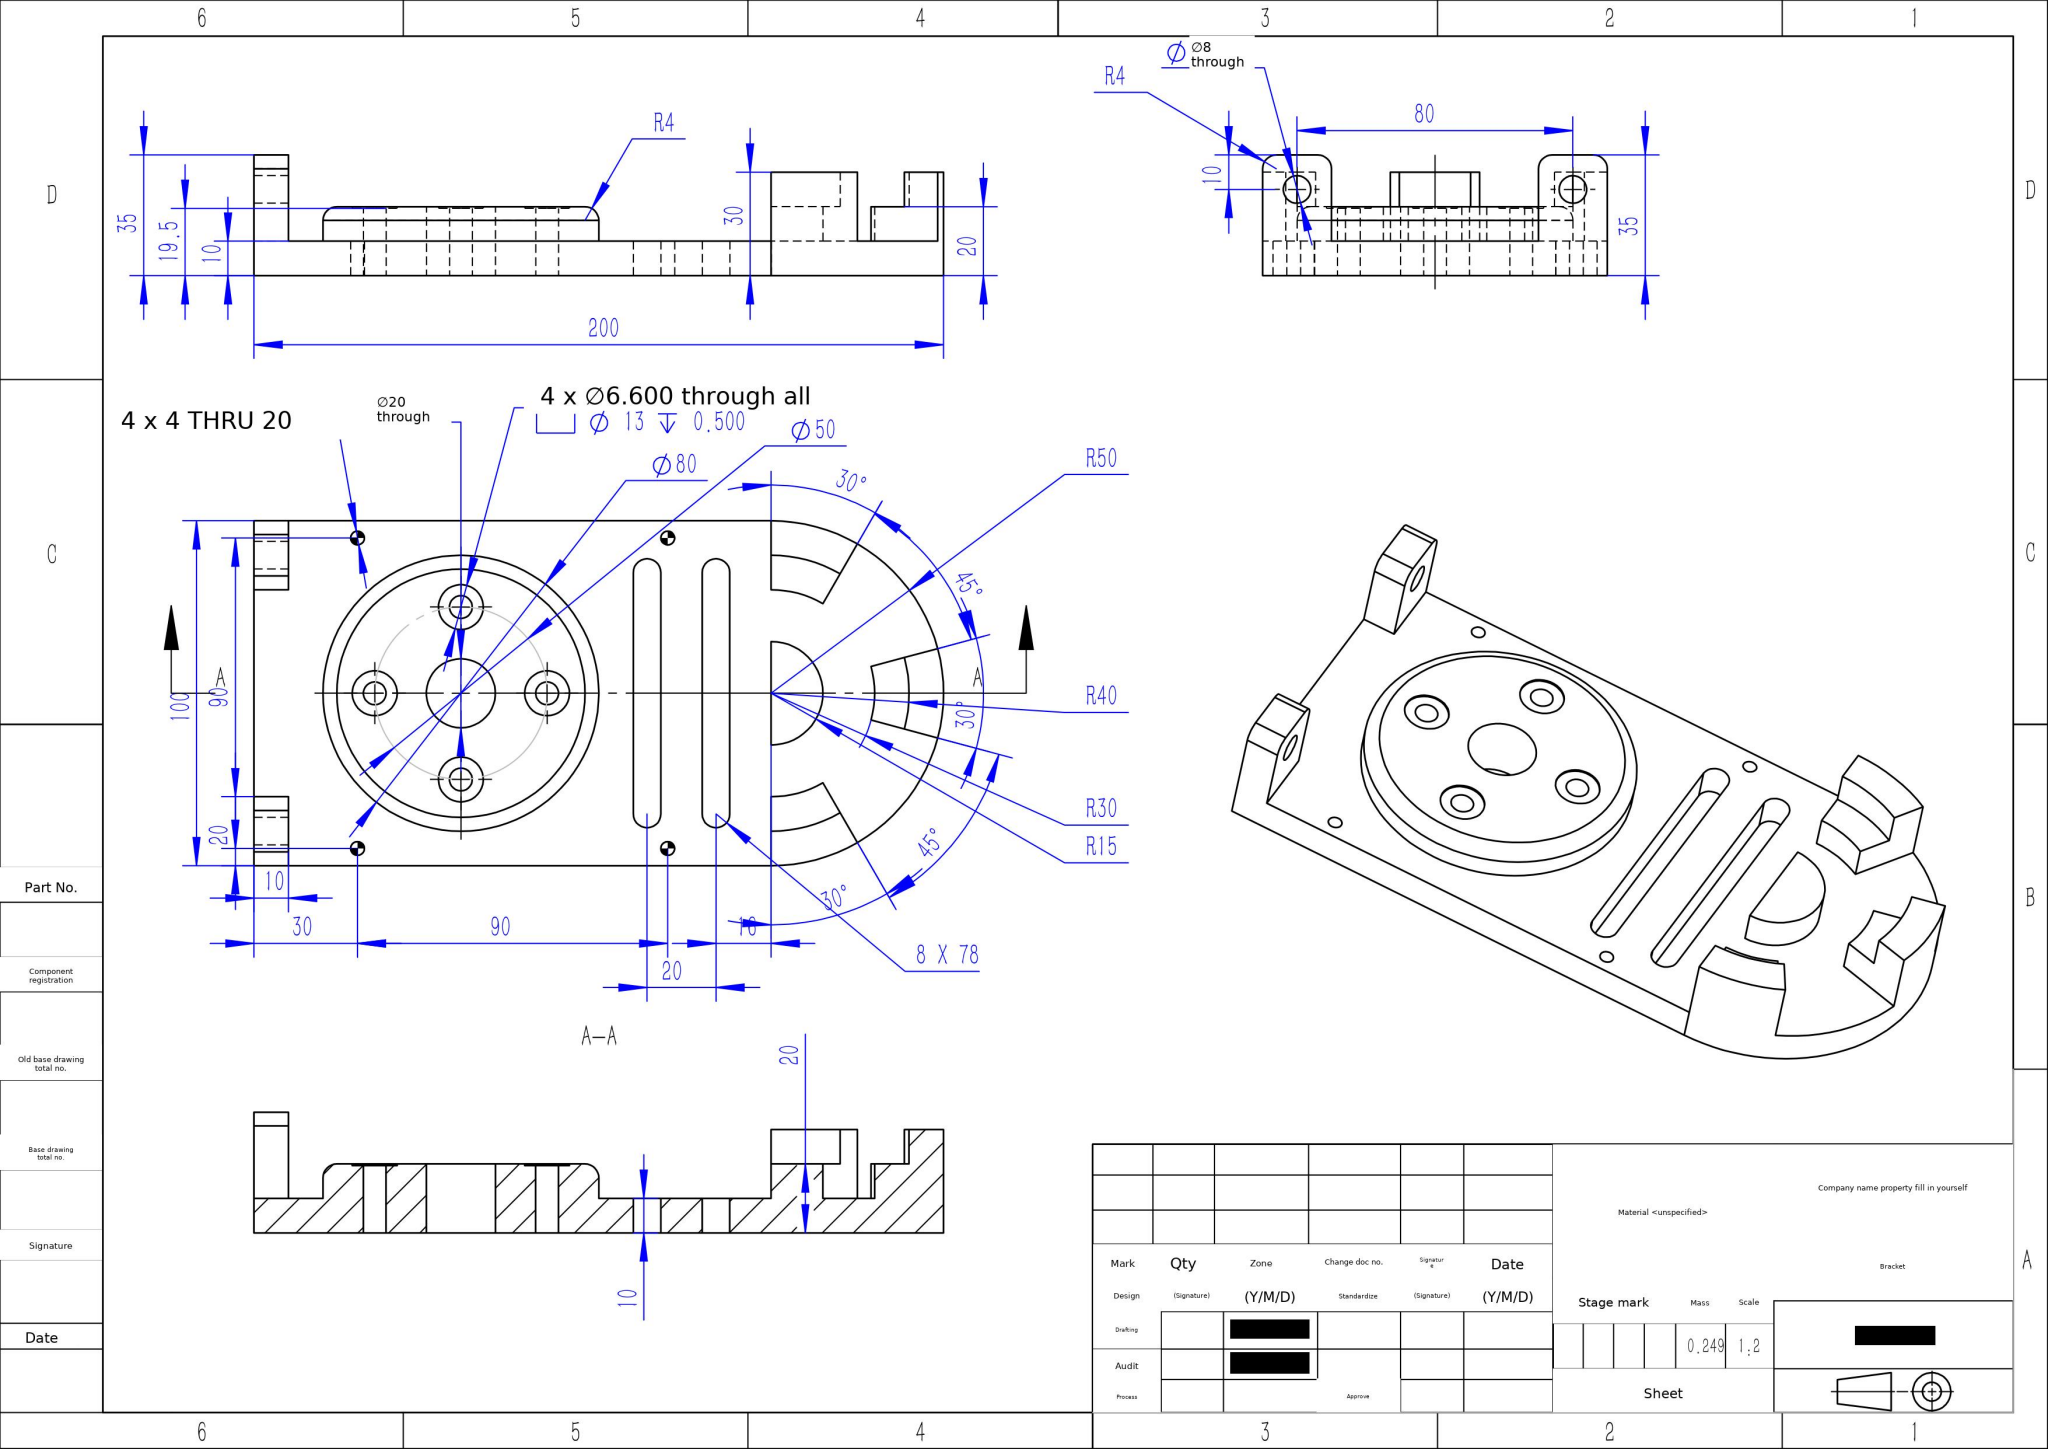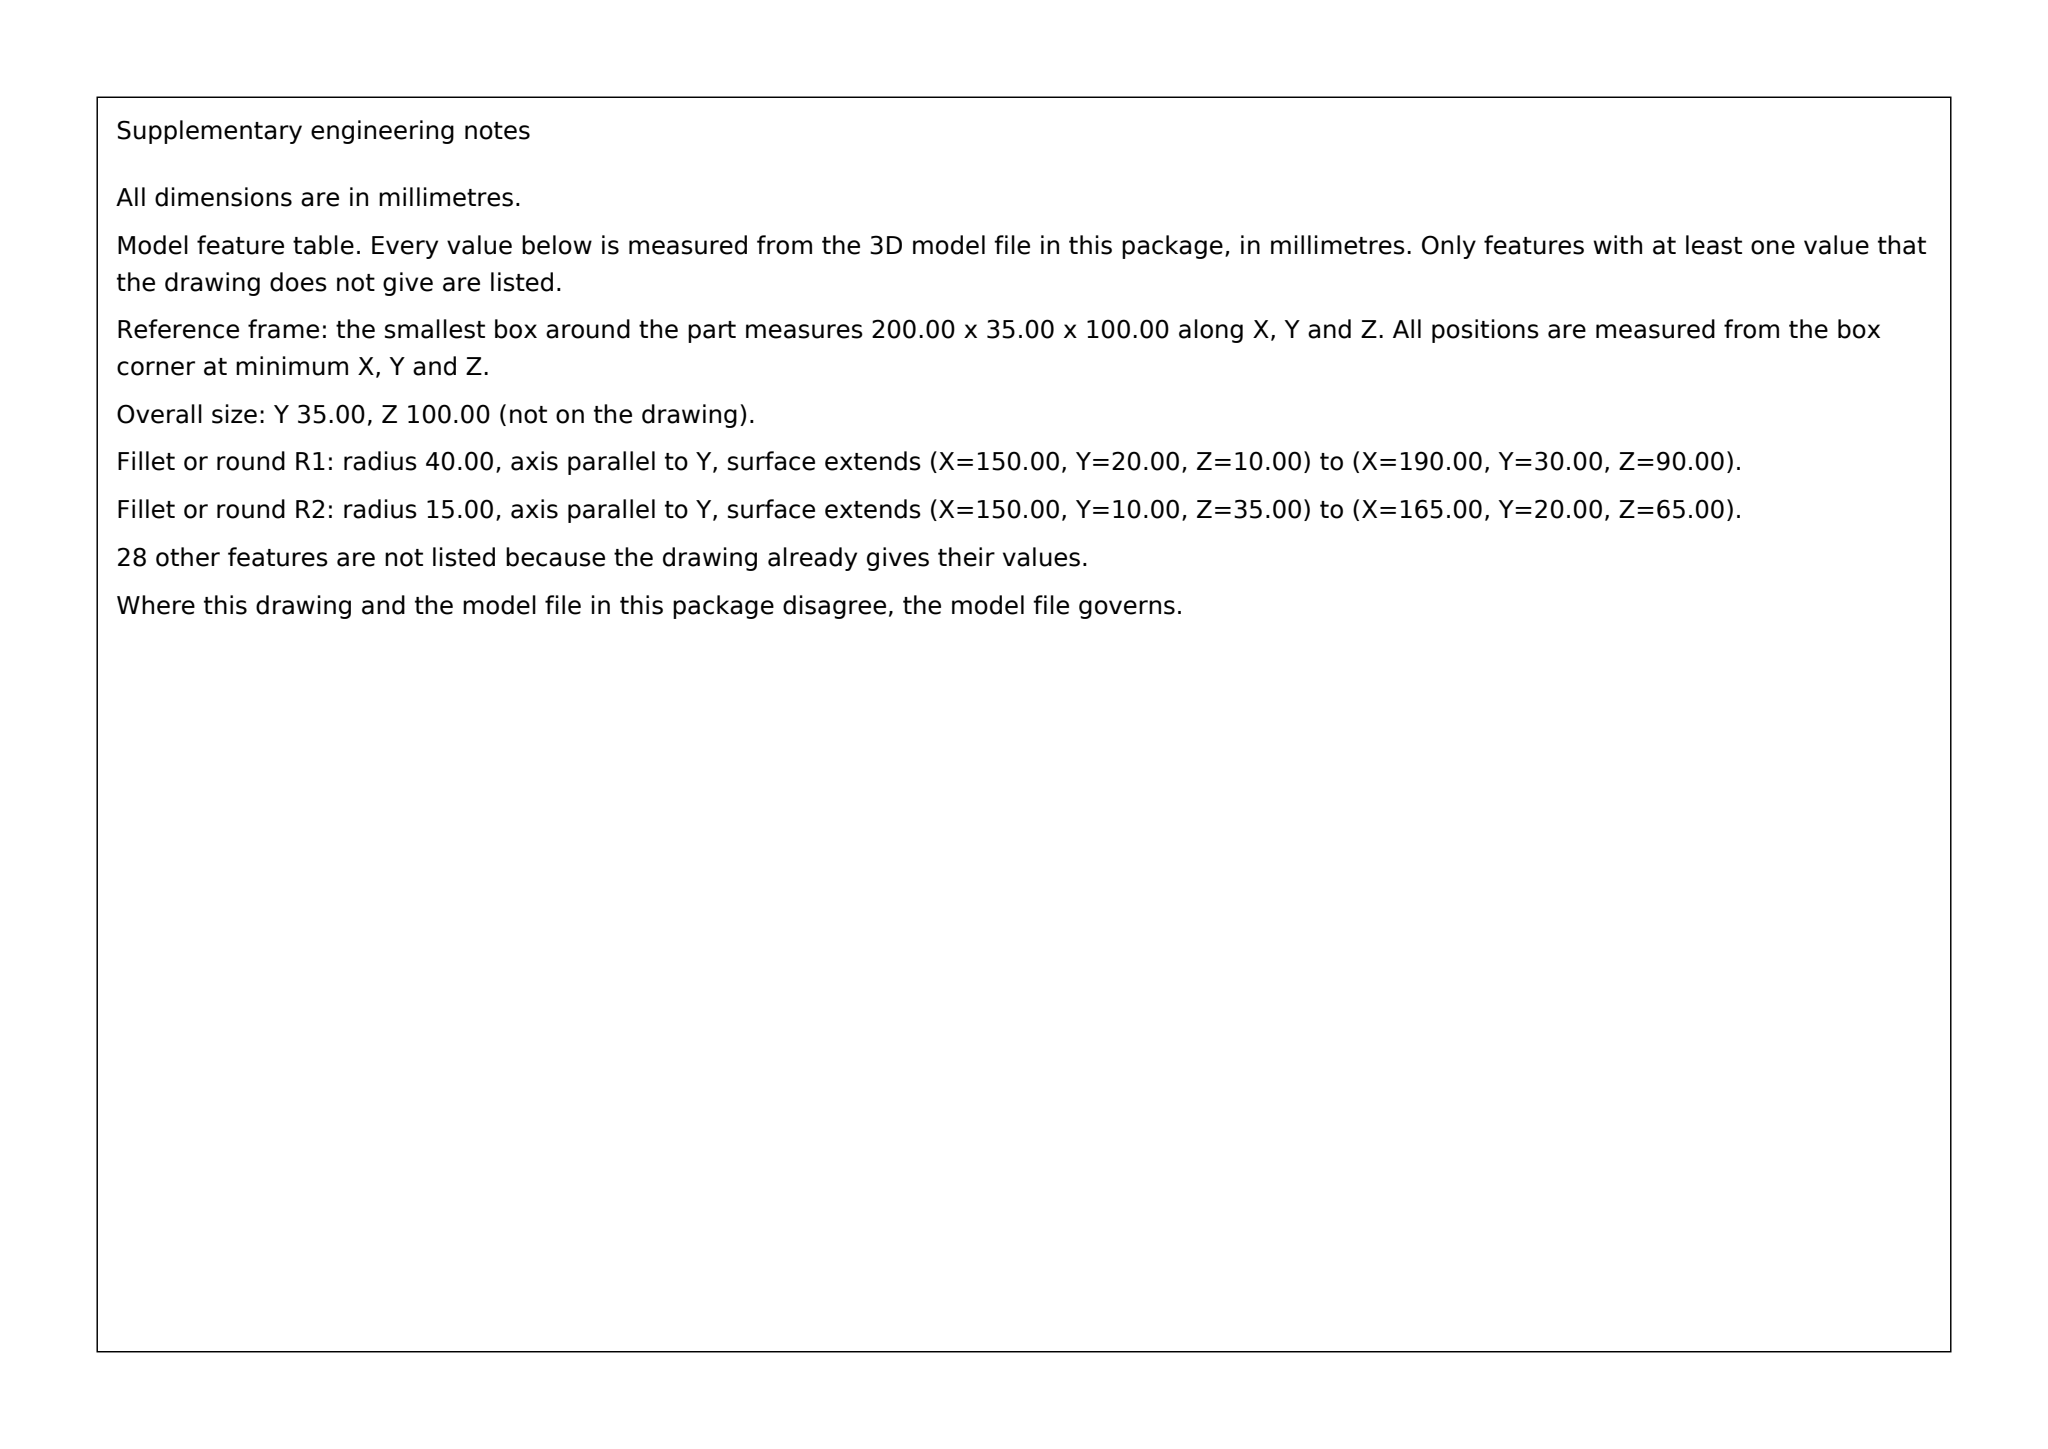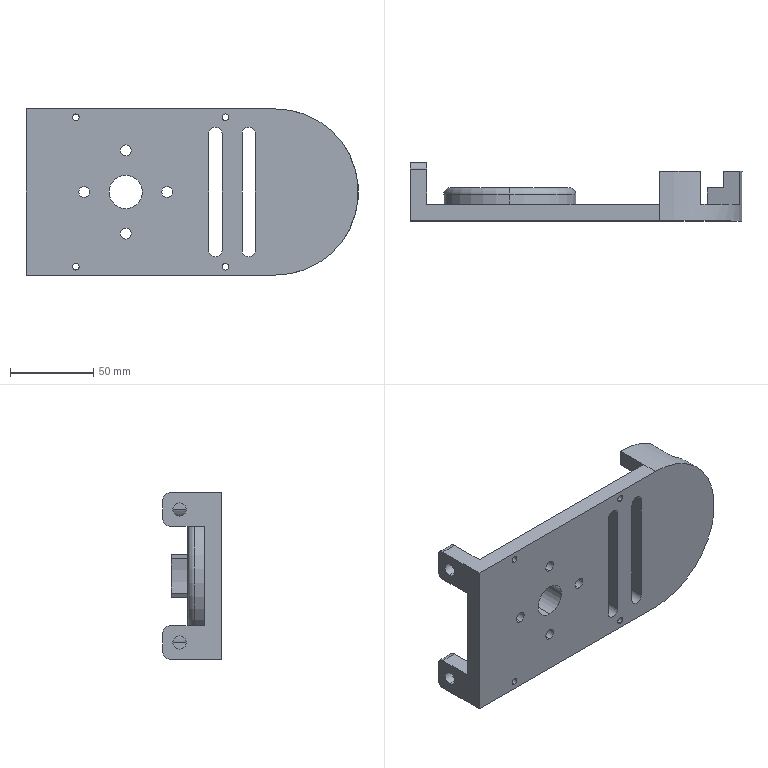Part | SolidWorks | mm | 1 solid | 86 faces | box 200 x 35 x 100 mm | volume 248793 mm3 | cylinder 50 | plane 34 | torus 2 | commonest cylinder face diameters 8 x14 4 x8 13 x8 6.6 x8 80 x5 60 x3 20 x2 30 x1